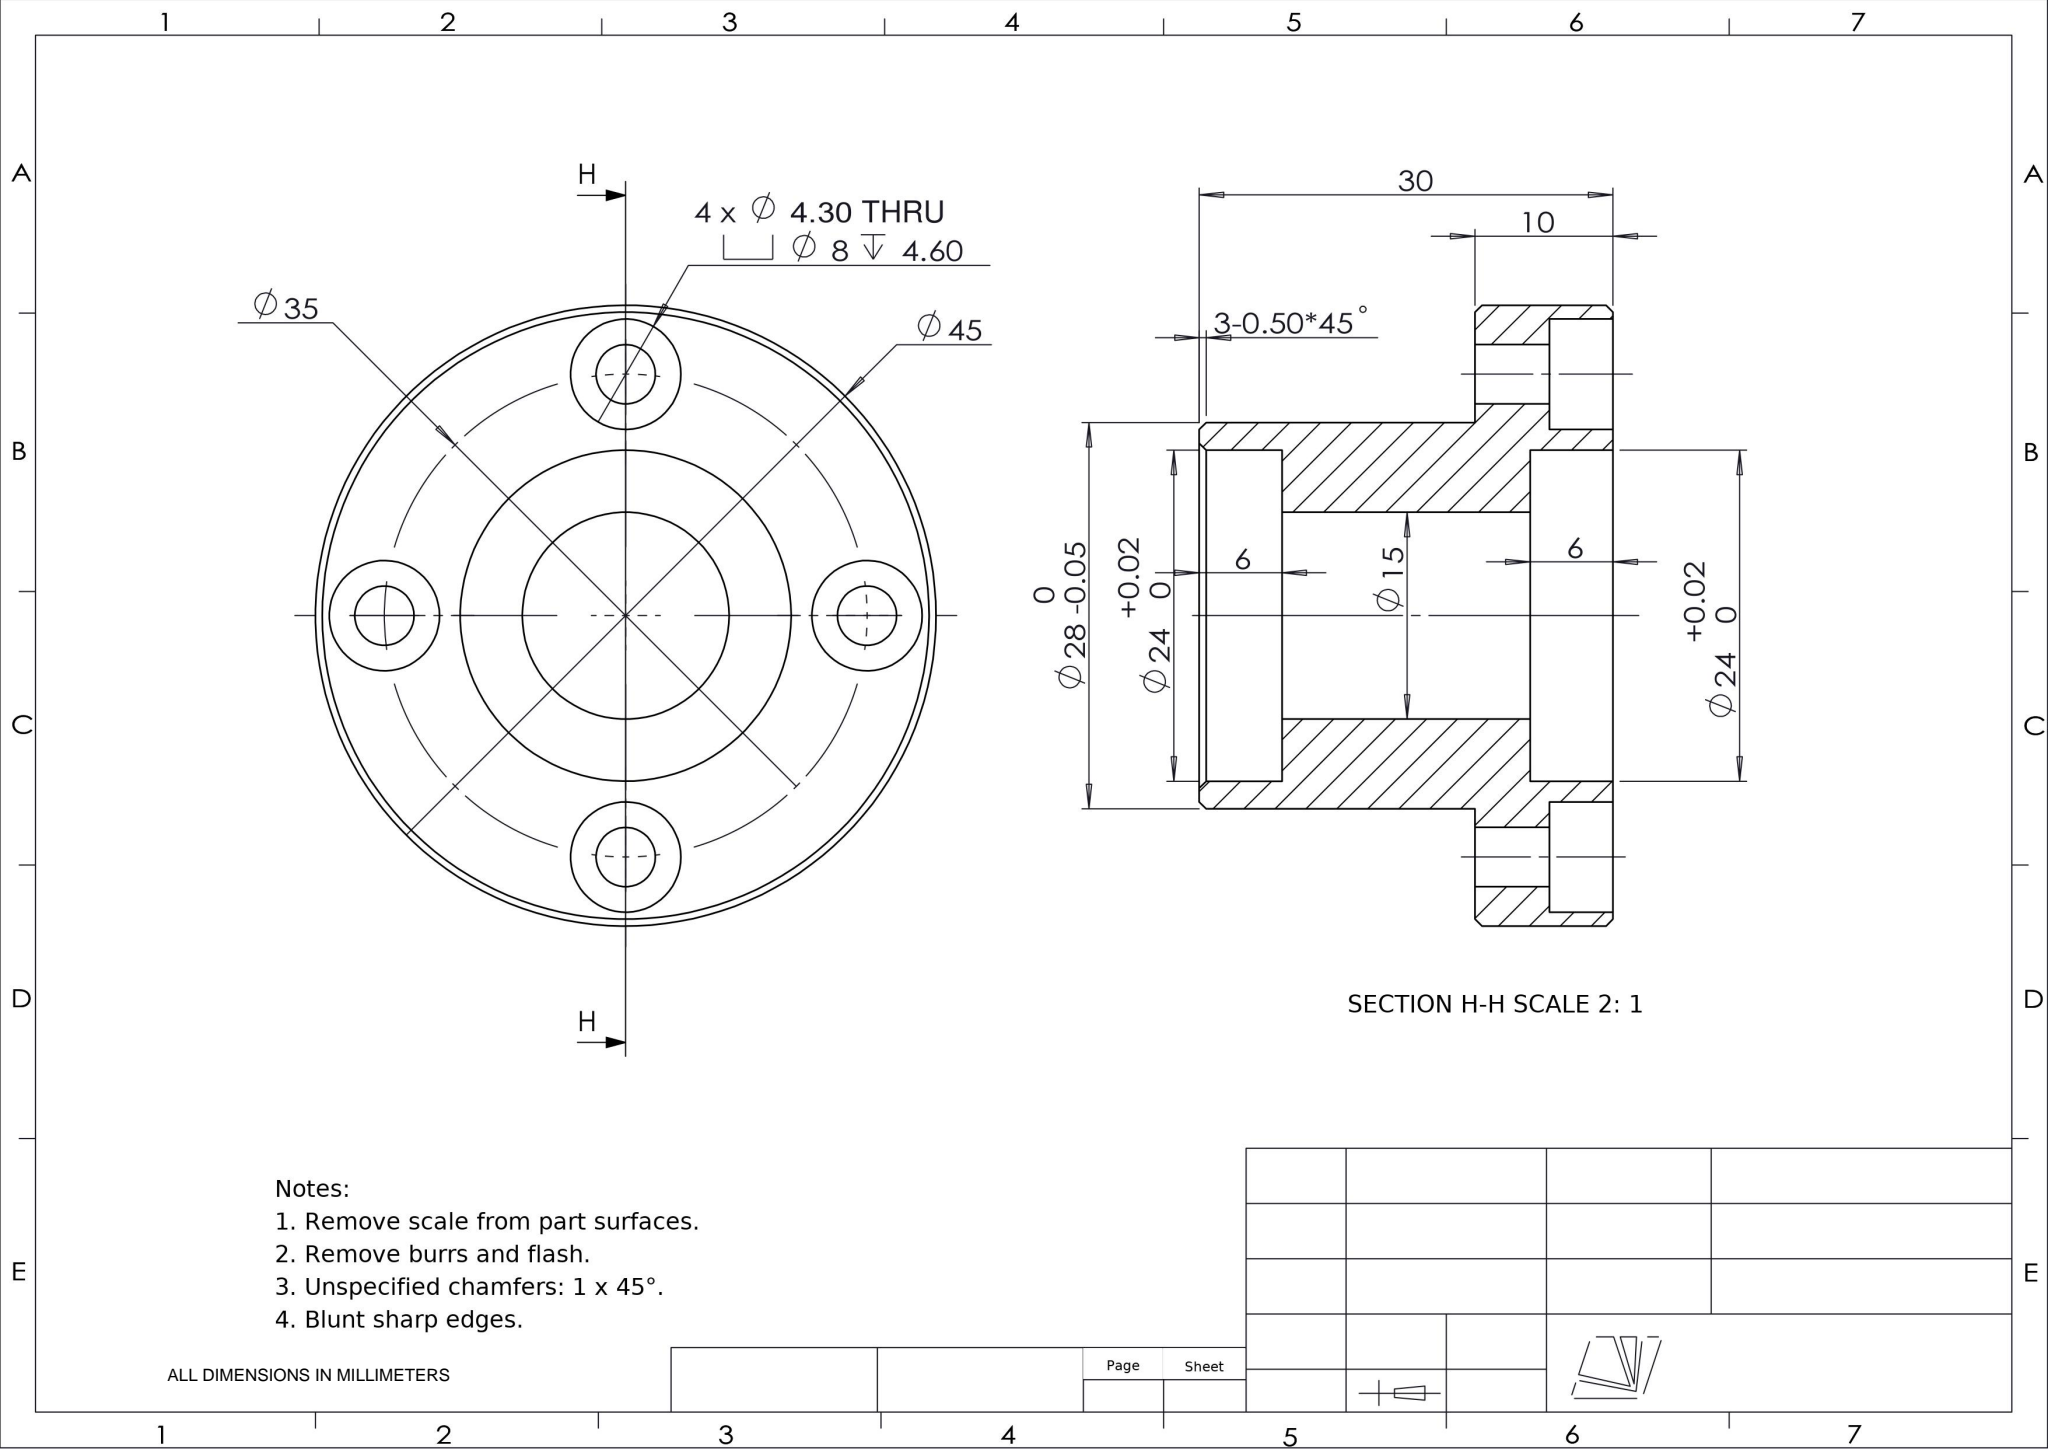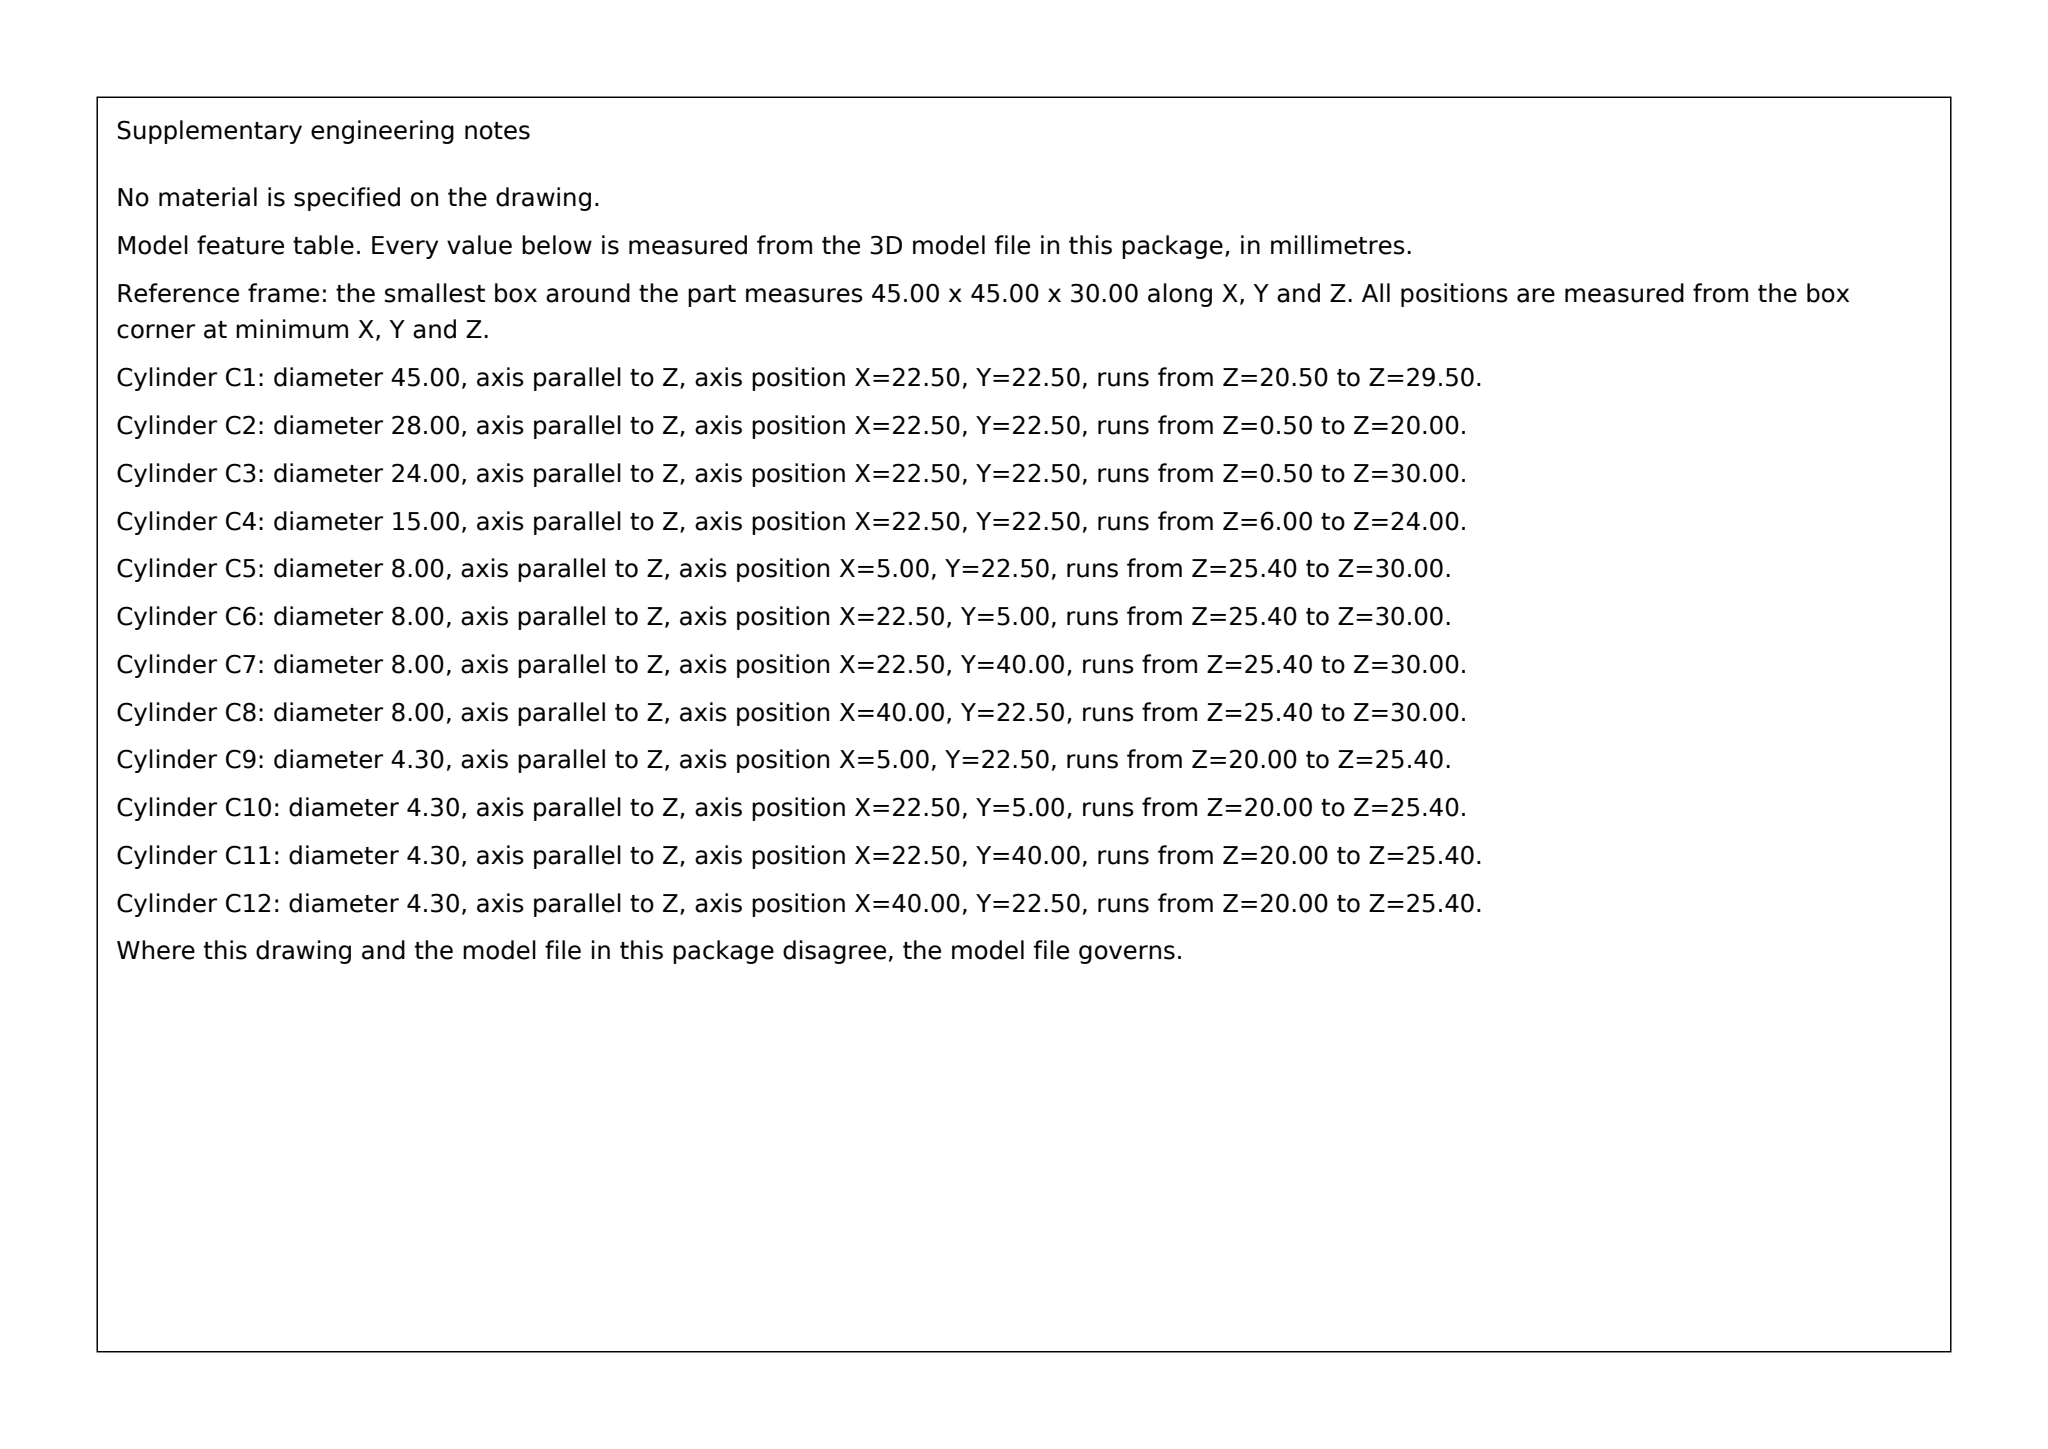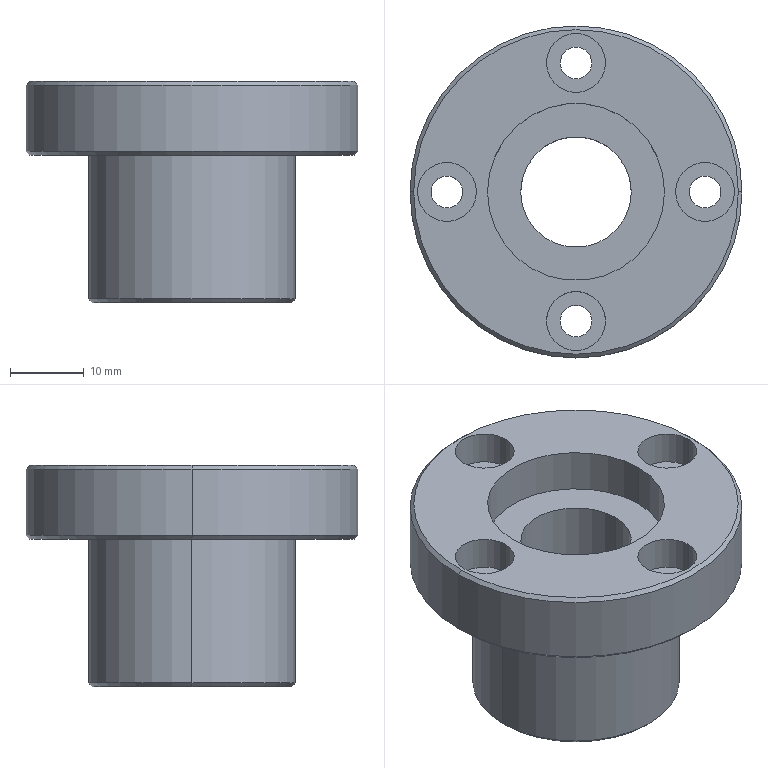Part | SolidWorks | mm | 1 solid | 43 faces | box 45 x 45 x 30 mm | volume 18316 mm3 | cylinder 26 | plane 9 | cone 8 | commonest cylinder face diameters 8 x8 4.3 x8 24 x4 28 x2 45 x2 15 x2
build123d program:
from build123d import *

# Parameters (mm, degrees)
SKETCH1_R                                            = 22.5
BOSS_EXTRUDE1_DEPTH                                  = 15
SKETCH2_R                                            = 7.5
CUT_EXTRUDE1_DEPTH                                   = 44.732
SKETCH3_R                                            = 12
CUT_EXTRUDE2_DEPTH                                   = 6
SKETCH5_R                                            = 30
SKETCH5_R_2                                          = 14
CUT_EXTRUDE3_DEPTH                                   = 38.583
HOLE_SIZE_ACCORDING_TO_THE_TYPE_OF_HEXAG_D           = 4.3
HOLE_SIZE_ACCORDING_TO_THE_TYPE_OF_HEXAG_CBORE_D     = 8
HOLE_SIZE_ACCORDING_TO_THE_TYPE_OF_HEXAG_CBORE_DEPTH = 4.6
CIRPATTERN1_COUNT                                    = 4
CHAMFER1_SIZE                                        = 0.5
CUT_EXTRUDE4_START                                   = -6
SKETCH8_R                                            = 12
CUT_EXTRUDE4_DEPTH                                   = 6
CHAMFER2_SIZE                                        = 0.5


with BuildPart() as part:
    # Sketch1 → Boss-Extrude1 (new, symmetric)
    with BuildSketch(Plane.XY):
        Circle(SKETCH1_R)
    extrude(amount=BOSS_EXTRUDE1_DEPTH, both=True)

    # Sketch2 → Cut-Extrude1 (cut, through all)
    with BuildSketch(Plane.XY.offset(15)):
        Circle(SKETCH2_R)
    extrude(amount=-CUT_EXTRUDE1_DEPTH, mode=Mode.SUBTRACT)

    # Sketch3 → Cut-Extrude2 (cut)
    with BuildSketch(Plane.XY.offset(15)):
        Circle(SKETCH3_R)
    extrude(amount=-CUT_EXTRUDE2_DEPTH, mode=Mode.SUBTRACT)

    # Sketch5 → Cut-Extrude3 (cut, through all)
    with BuildSketch(Plane.XY.offset(5)):
        Circle(SKETCH5_R)
        Circle(SKETCH5_R_2, mode=Mode.SUBTRACT)
    extrude(amount=-CUT_EXTRUDE3_DEPTH, mode=Mode.SUBTRACT)

    # Hole Size according to the type of Hexag (through all)
    with Locations(Plane.XY.offset(15)):
        with Locations((0, 17.5)):
            hole_size_according_to_the_type_of_hexag = CounterBoreHole(HOLE_SIZE_ACCORDING_TO_THE_TYPE_OF_HEXAG_D / 2, HOLE_SIZE_ACCORDING_TO_THE_TYPE_OF_HEXAG_CBORE_D / 2, HOLE_SIZE_ACCORDING_TO_THE_TYPE_OF_HEXAG_CBORE_DEPTH)

    # CirPattern1: Hole Size according to the type of Hexag ×4 about axis
    cirpattern1_axis = Axis((0, 0, 0), (0, 0, 1))
    for i in range(1, CIRPATTERN1_COUNT):
        add(hole_size_according_to_the_type_of_hexag.rotate(cirpattern1_axis, i * 360 / CIRPATTERN1_COUNT), mode=Mode.SUBTRACT)

    # Chamfer1
    chamfer1_edges = [part.edges().sort_by_distance(p)[0] for p in [
        (-22.5, 0, 5),
        (-22.5, 0, 15),
    ]]
    chamfer(chamfer1_edges, length=CHAMFER1_SIZE)

    # Sketch8 → Cut-Extrude4 (cut)
    with BuildSketch(Plane(origin=(0, 0, -15), x_dir=(-1, 0, 0), z_dir=(0, 0, -1)).offset(CUT_EXTRUDE4_START)):
        with Locations(Location((0, 0, 0), (0, 0, 180))):
            Circle(SKETCH8_R)
    extrude(amount=CUT_EXTRUDE4_DEPTH, mode=Mode.SUBTRACT)

    # Chamfer2
    chamfer2_edges = [part.edges().sort_by_distance(p)[0] for p in [
        (-14, 0, -15),
        (-12, 0, -15),
    ]]
    chamfer(chamfer2_edges, length=CHAMFER2_SIZE)


solid = part.part